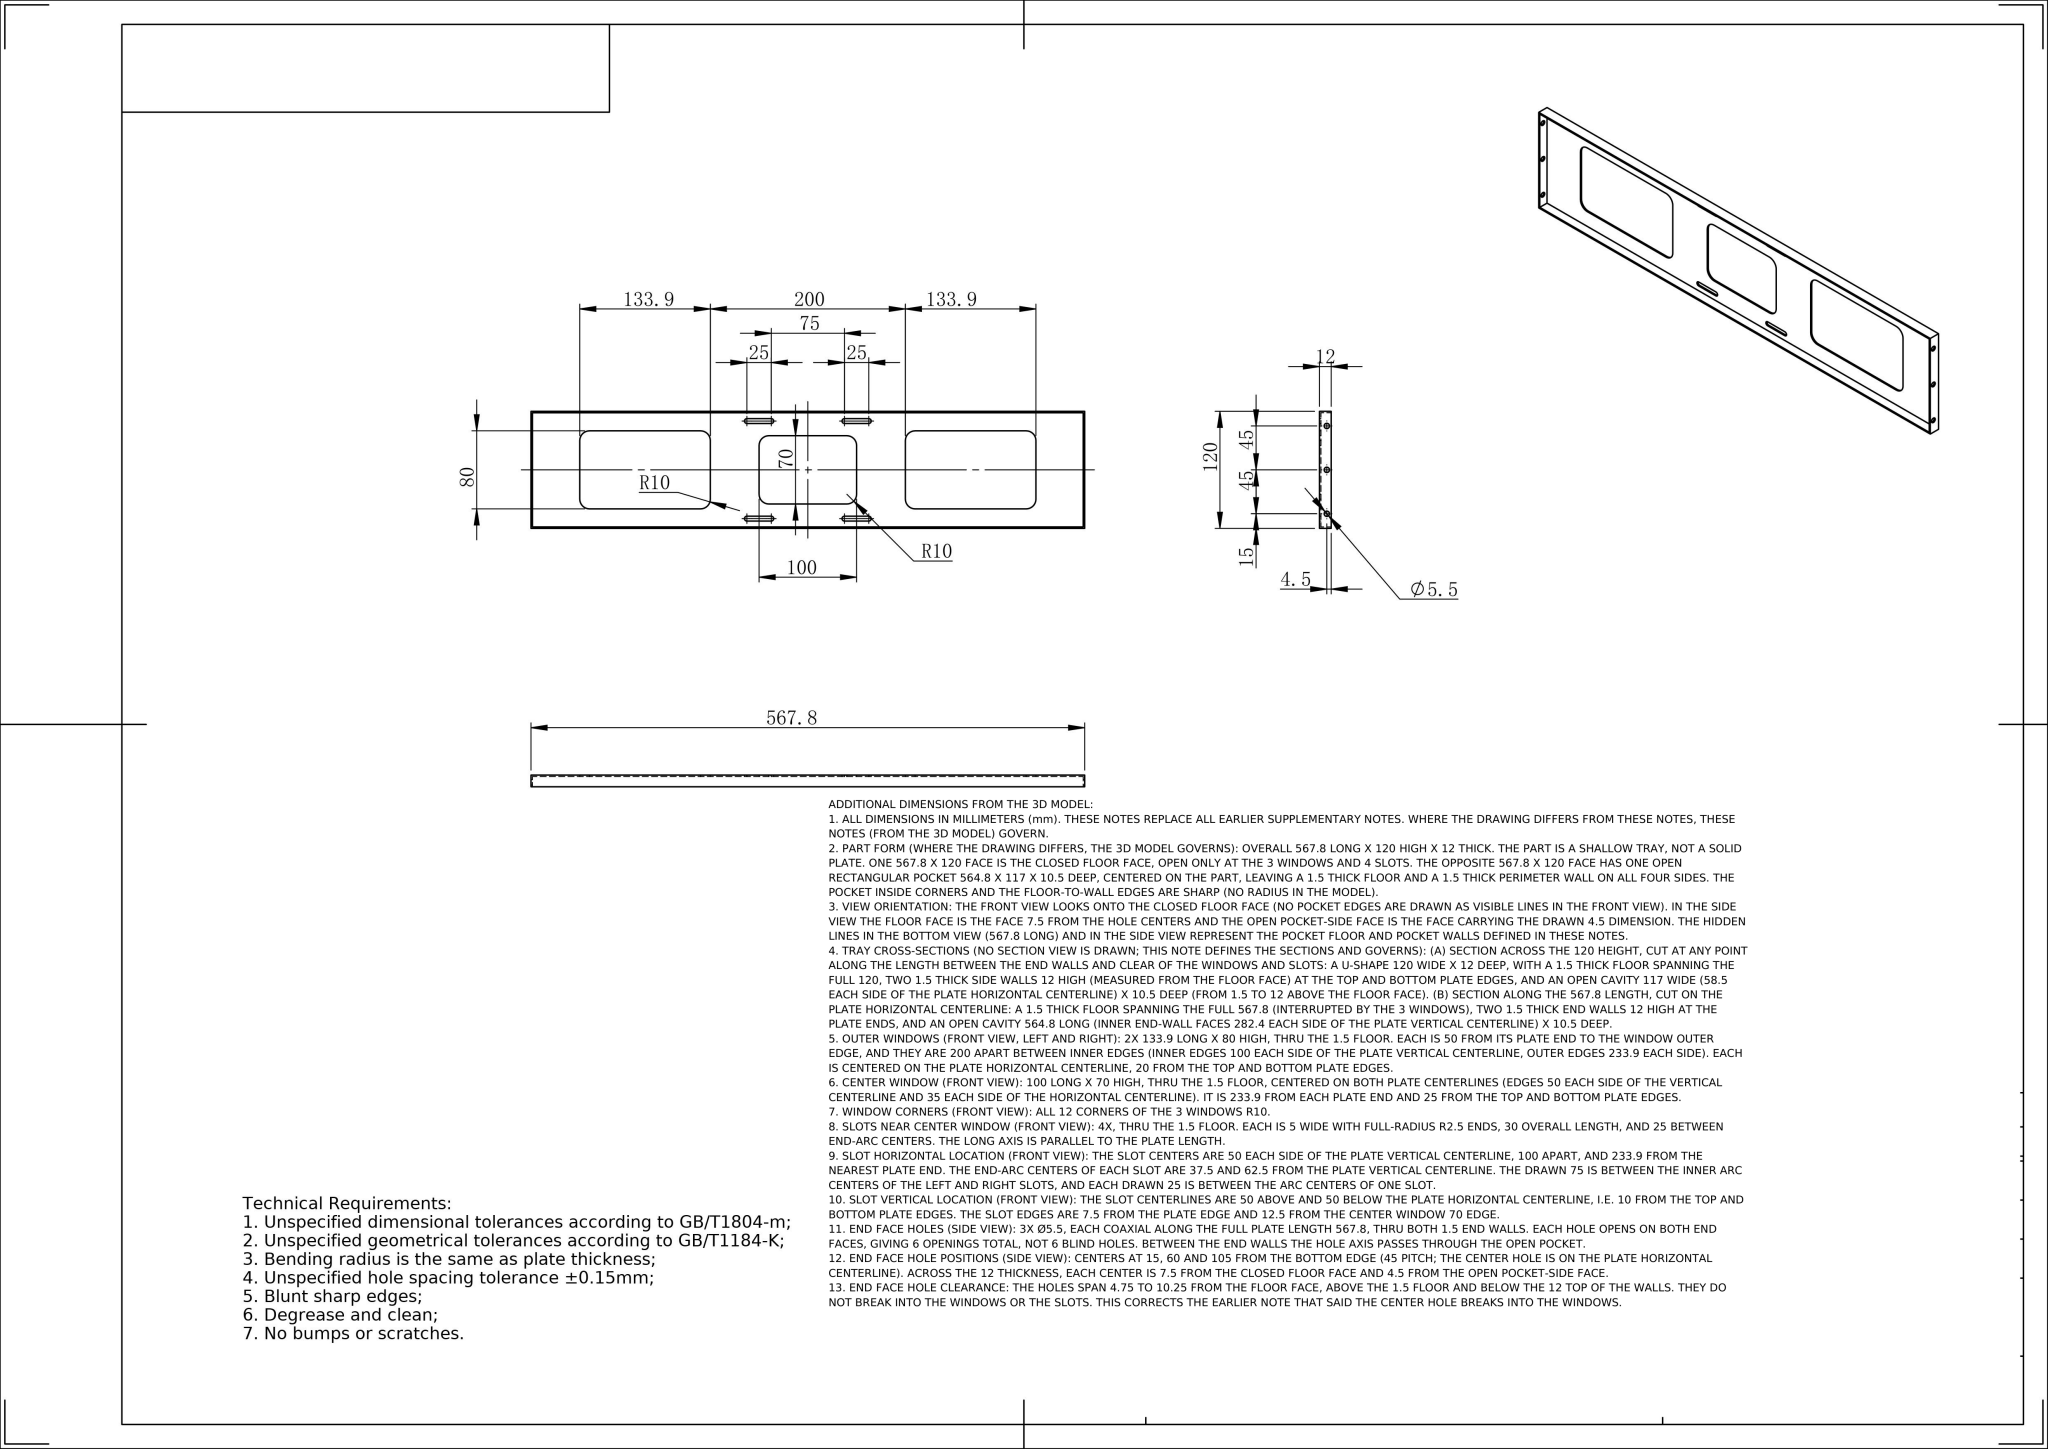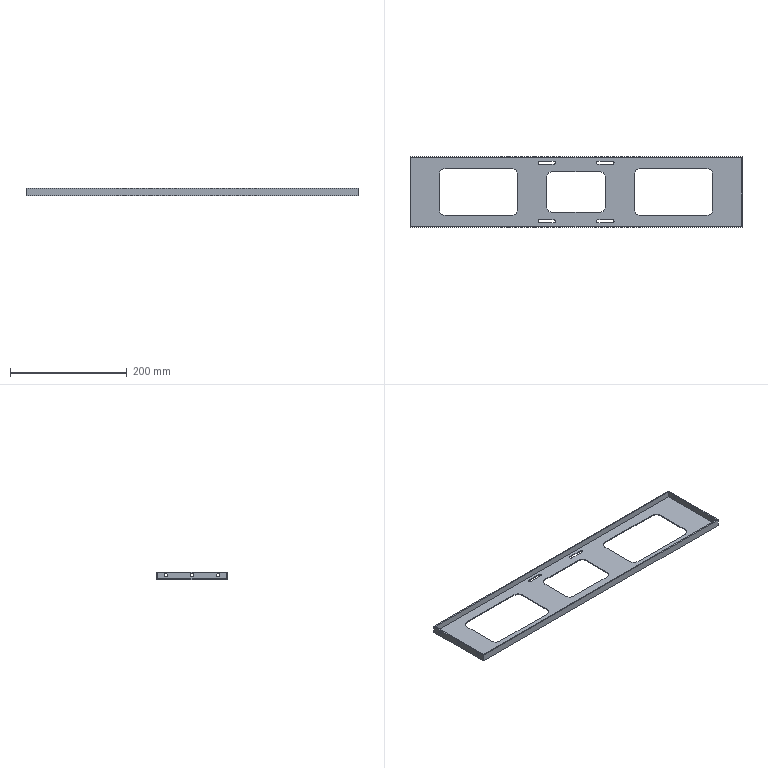Part | NX | mm | 1 solid | 67 faces | box 567.8 x 120 x 12 mm | volume 80444 mm3 | cylinder 36 | plane 31 | commonest cylinder face diameters 5.5 x12 5 x12 20 x12